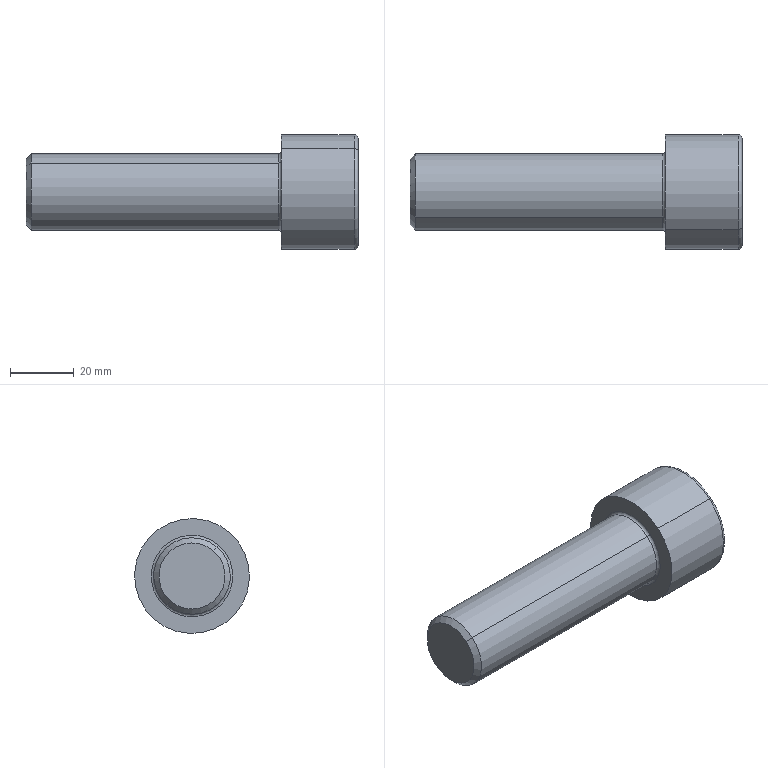Component | SolidWorks | socket head cap screw_iso-3 | 1 solid | 27 faces | box 104 x 36 x 36 mm | volume 55912 mm3 | plane 15 | cone 4 | torus 4 | cylinder 4 | commonest cylinder face diameters 24 x2 36 x2
STEP:
#1=COLOUR_RGB('',0.7922,0.8196,0.9333);
#2=FILL_AREA_STYLE_COLOUR('',#1);
#3=FILL_AREA_STYLE('',(#2));
#4=SURFACE_STYLE_FILL_AREA(#3);
#5=SURFACE_SIDE_STYLE('',(#4));
#6=SURFACE_STYLE_USAGE(.BOTH.,#5);
#7=PRESENTATION_STYLE_ASSIGNMENT((#6));
#8=CARTESIAN_POINT('',(-2.092,1.23,0.6693));
#9=VERTEX_POINT('',#8);
#10=CARTESIAN_POINT('',(-1.873,1.478,0.3823));
#11=VERTEX_POINT('',#10);
#12=CARTESIAN_POINT('',(-1.873,1.478,0.3823));
#13=DIRECTION('',(0.5,0.5664,-0.6551));
#14=VECTOR('',#13,39.37);
#15=LINE('',#12,#14);
#16=EDGE_CURVE('',#9,#11,#15,.T.);
#17=ORIENTED_EDGE('',*,*,#16,.F.);
#18=CARTESIAN_POINT('',(-1.873,0.9822,0.9563));
#19=VERTEX_POINT('',#18);
#20=CARTESIAN_POINT('',(-1.873,0.9822,0.9563));
#21=DIRECTION('',(0.5,-0.5664,0.6551));
#22=VECTOR('',#21,39.37);
#23=LINE('',#20,#22);
#24=EDGE_CURVE('',#9,#19,#23,.T.);
#25=ORIENTED_EDGE('',*,*,#24,.T.);
#26=CARTESIAN_POINT('',(-1.873,0.8577,0.5979));
#27=VERTEX_POINT('',#26);
#28=CARTESIAN_POINT('',(-1.873,1.23,0.6693));
#29=DIRECTION('',(1.,0.,-0.));
#30=DIRECTION('',(0.,0.654,-0.7565));
#31=AXIS2_PLACEMENT_3D('',#28,#29,#30);
#32=CIRCLE('',#31,0.3794);
#33=EDGE_CURVE('',#19,#27,#32,.T.);
#34=ORIENTED_EDGE('',*,*,#33,.T.);
#35=CARTESIAN_POINT('',(-1.873,1.106,0.3109));
#36=VERTEX_POINT('',#35);
#37=CARTESIAN_POINT('',(-1.873,1.23,0.6693));
#38=DIRECTION('',(1.,0.,-0.));
#39=DIRECTION('',(0.,0.654,-0.7565));
#40=AXIS2_PLACEMENT_3D('',#37,#38,#39);
#41=CIRCLE('',#40,0.3794);
#42=EDGE_CURVE('',#27,#36,#41,.T.);
#43=ORIENTED_EDGE('',*,*,#42,.T.);
#44=CARTESIAN_POINT('',(-1.873,1.23,0.6693));
#45=DIRECTION('',(1.,0.,-0.));
#46=DIRECTION('',(0.,0.654,-0.7565));
#47=AXIS2_PLACEMENT_3D('',#44,#45,#46);
#48=CIRCLE('',#47,0.3794);
#49=EDGE_CURVE('',#36,#11,#48,.T.);
#50=ORIENTED_EDGE('',*,*,#49,.T.);
#51=EDGE_LOOP('',(#17,#25,#34,#43,#50));
#52=FACE_OUTER_BOUND('',#51,.T.);
#53=CARTESIAN_POINT('',(-1.873,1.23,0.6693));
#54=DIRECTION('',(1.,0.,-0.));
#55=DIRECTION('',(0.,0.654,-0.7565));
#56=AXIS2_PLACEMENT_3D('',#53,#54,#55);
#57=CONICAL_SURFACE('',#56,0.3794,1.047);
#58=ADVANCED_FACE('',(#52),#57,.F.);
#59=CARTESIAN_POINT('',(-1.425,0.7668,1.205));
#60=VERTEX_POINT('',#59);
#61=CARTESIAN_POINT('',(-1.425,1.694,0.1332));
#62=VERTEX_POINT('',#61);
#63=CARTESIAN_POINT('',(-1.425,1.23,0.6693));
#64=DIRECTION('',(-1.,-0.,0.));
#65=DIRECTION('',(0.,0.654,-0.7565));
#66=AXIS2_PLACEMENT_3D('',#63,#64,#65);
#67=CIRCLE('',#66,0.7087);
#68=EDGE_CURVE('',#60,#62,#67,.T.);
#69=ORIENTED_EDGE('',*,*,#68,.F.);
#70=CARTESIAN_POINT('',(-1.378,0.7977,1.17));
#71=VERTEX_POINT('',#70);
#72=CARTESIAN_POINT('',(-1.425,0.7977,1.17));
#73=DIRECTION('',(-0.,0.7565,0.654));
#74=DIRECTION('',(0.,-0.654,0.7565));
#75=AXIS2_PLACEMENT_3D('',#72,#73,#74);
#76=CIRCLE('',#75,0.04724);
#77=EDGE_CURVE('',#60,#71,#76,.T.);
#78=ORIENTED_EDGE('',*,*,#77,.T.);
#79=CARTESIAN_POINT('',(-1.378,1.663,0.169));
#80=VERTEX_POINT('',#79);
#81=CARTESIAN_POINT('',(-1.378,1.23,0.6693));
#82=DIRECTION('',(1.,0.,-0.));
#83=DIRECTION('',(0.,0.654,-0.7565));
#84=AXIS2_PLACEMENT_3D('',#81,#82,#83);
#85=CIRCLE('',#84,0.6614);
#86=EDGE_CURVE('',#80,#71,#85,.T.);
#87=ORIENTED_EDGE('',*,*,#86,.F.);
#88=CARTESIAN_POINT('',(-1.425,1.663,0.169));
#89=DIRECTION('',(0.,-0.7565,-0.654));
#90=DIRECTION('',(0.,0.654,-0.7565));
#91=AXIS2_PLACEMENT_3D('',#88,#89,#90);
#92=CIRCLE('',#91,0.04724);
#93=EDGE_CURVE('',#62,#80,#92,.T.);
#94=ORIENTED_EDGE('',*,*,#93,.F.);
#95=EDGE_LOOP('',(#69,#78,#87,#94));
#96=FACE_OUTER_BOUND('',#95,.T.);
#97=CARTESIAN_POINT('',(-1.425,1.23,0.6693));
#98=DIRECTION('',(1.,0.,-0.));
#99=DIRECTION('',(-0.,0.654,-0.7565));
#100=AXIS2_PLACEMENT_3D('',#97,#98,#99);
#101=TOROIDAL_SURFACE('',#100,0.6614,0.04724);
#102=ADVANCED_FACE('',(#96),#101,.T.);
#103=CARTESIAN_POINT('',(-2.354,1.539,0.3119));
#104=VERTEX_POINT('',#103);
#105=CARTESIAN_POINT('',(-2.354,0.9213,1.027));
#106=VERTEX_POINT('',#105);
#107=CARTESIAN_POINT('',(-2.354,1.23,0.6693));
#108=DIRECTION('',(-1.,-0.,0.));
#109=DIRECTION('',(0.,-0.654,0.7565));
#110=AXIS2_PLACEMENT_3D('',#107,#108,#109);
#111=CIRCLE('',#110,0.4724);
#112=EDGE_CURVE('',#104,#106,#111,.T.);
#113=ORIENTED_EDGE('',*,*,#112,.F.);
#114=CARTESIAN_POINT('',(-2.323,1.56,0.2881));
#115=VERTEX_POINT('',#114);
#116=CARTESIAN_POINT('',(-2.354,1.56,0.2881));
#117=DIRECTION('',(-0.,0.7565,0.654));
#118=DIRECTION('',(0.,-0.654,0.7565));
#119=AXIS2_PLACEMENT_3D('',#116,#117,#118);
#120=CIRCLE('',#119,0.0315);
#121=EDGE_CURVE('',#104,#115,#120,.T.);
#122=ORIENTED_EDGE('',*,*,#121,.T.);
#123=CARTESIAN_POINT('',(-2.323,0.9007,1.051));
#124=VERTEX_POINT('',#123);
#125=CARTESIAN_POINT('',(-2.323,1.23,0.6693));
#126=DIRECTION('',(1.,0.,-0.));
#127=DIRECTION('',(0.,-0.654,0.7565));
#128=AXIS2_PLACEMENT_3D('',#125,#126,#127);
#129=CIRCLE('',#128,0.5039);
#130=EDGE_CURVE('',#124,#115,#129,.T.);
#131=ORIENTED_EDGE('',*,*,#130,.F.);
#132=CARTESIAN_POINT('',(-2.354,0.9007,1.051));
#133=DIRECTION('',(0.,-0.7565,-0.654));
#134=DIRECTION('',(0.,0.654,-0.7565));
#135=AXIS2_PLACEMENT_3D('',#132,#133,#134);
#136=CIRCLE('',#135,0.0315);
#137=EDGE_CURVE('',#106,#124,#136,.T.);
#138=ORIENTED_EDGE('',*,*,#137,.F.);
#139=EDGE_LOOP('',(#113,#122,#131,#138));
#140=FACE_OUTER_BOUND('',#139,.T.);
#141=CARTESIAN_POINT('',(-2.354,1.23,0.6693));
#142=DIRECTION('',(-1.,-0.,0.));
#143=DIRECTION('',(0.,-0.654,0.7565));
#144=AXIS2_PLACEMENT_3D('',#141,#142,#143);
#145=TOROIDAL_SURFACE('',#144,0.5039,0.0315);
#146=ADVANCED_FACE('',(#140),#145,.F.);
#147=CARTESIAN_POINT('',(-5.472,1.497,0.361));
#148=VERTEX_POINT('',#147);
#149=CARTESIAN_POINT('',(-5.472,0.9638,0.9776));
#150=VERTEX_POINT('',#149);
#151=CARTESIAN_POINT('',(-5.472,1.23,0.6693));
#152=DIRECTION('',(1.,0.,-0.));
#153=DIRECTION('',(0.,0.654,-0.7565));
#154=AXIS2_PLACEMENT_3D('',#151,#152,#153);
#155=CIRCLE('',#154,0.4076);
#156=EDGE_CURVE('',#148,#150,#155,.T.);
#157=ORIENTED_EDGE('',*,*,#156,.T.);
#158=CARTESIAN_POINT('',(-5.408,0.9213,1.027));
#159=VERTEX_POINT('',#158);
#160=CARTESIAN_POINT('',(-5.472,0.9638,0.9776));
#161=DIRECTION('',(0.7071,-0.4625,0.5349));
#162=VECTOR('',#161,39.37);
#163=LINE('',#160,#162);
#164=EDGE_CURVE('',#150,#159,#163,.T.);
#165=ORIENTED_EDGE('',*,*,#164,.T.);
#166=CARTESIAN_POINT('',(-5.408,1.539,0.3119));
#167=VERTEX_POINT('',#166);
#168=CARTESIAN_POINT('',(-5.408,1.23,0.6693));
#169=DIRECTION('',(1.,0.,-0.));
#170=DIRECTION('',(0.,0.654,-0.7565));
#171=AXIS2_PLACEMENT_3D('',#168,#169,#170);
#172=CIRCLE('',#171,0.4724);
#173=EDGE_CURVE('',#167,#159,#172,.T.);
#174=ORIENTED_EDGE('',*,*,#173,.F.);
#175=CARTESIAN_POINT('',(-5.472,1.497,0.361));
#176=DIRECTION('',(0.7071,0.4625,-0.5349));
#177=VECTOR('',#176,39.37);
#178=LINE('',#175,#177);
#179=EDGE_CURVE('',#148,#167,#178,.T.);
#180=ORIENTED_EDGE('',*,*,#179,.F.);
#181=EDGE_LOOP('',(#157,#165,#174,#180));
#182=FACE_OUTER_BOUND('',#181,.T.);
#183=CARTESIAN_POINT('',(-5.472,1.23,0.6693));
#184=DIRECTION('',(1.,0.,-0.));
#185=DIRECTION('',(0.,0.654,-0.7565));
#186=AXIS2_PLACEMENT_3D('',#183,#184,#185);
#187=CONICAL_SURFACE('',#186,0.4076,0.7854);
#188=ADVANCED_FACE('',(#182),#187,.T.);
#189=ORIENTED_EDGE('',*,*,#173,.T.);
#190=CARTESIAN_POINT('',(-0.128,0.9213,1.027));
#191=DIRECTION('',(1.,0.,-0.));
#192=VECTOR('',#191,39.37);
#193=LINE('',#190,#192);
#194=EDGE_CURVE('',#159,#106,#193,.T.);
#195=ORIENTED_EDGE('',*,*,#194,.T.);
#196=CARTESIAN_POINT('',(-2.354,1.23,0.6693));
#197=DIRECTION('',(-1.,-0.,0.));
#198=DIRECTION('',(0.,-0.654,0.7565));
#199=AXIS2_PLACEMENT_3D('',#196,#197,#198);
#200=CIRCLE('',#199,0.4724);
#201=EDGE_CURVE('',#106,#104,#200,.T.);
#202=ORIENTED_EDGE('',*,*,#201,.T.);
#203=CARTESIAN_POINT('',(-0.128,1.539,0.3119));
#204=DIRECTION('',(1.,0.,-0.));
#205=VECTOR('',#204,39.37);
#206=LINE('',#203,#205);
#207=EDGE_CURVE('',#167,#104,#206,.T.);
#208=ORIENTED_EDGE('',*,*,#207,.F.);
#209=EDGE_LOOP('',(#189,#195,#202,#208));
#210=FACE_OUTER_BOUND('',#209,.T.);
#211=CARTESIAN_POINT('',(-0.128,1.23,0.6693));
#212=DIRECTION('',(1.,0.,-0.));
#213=DIRECTION('',(0.,0.654,-0.7565));
#214=AXIS2_PLACEMENT_3D('',#211,#212,#213);
#215=CYLINDRICAL_SURFACE('',#214,0.4724);
#216=ADVANCED_FACE('',(#210),#215,.T.);
#217=CARTESIAN_POINT('',(-2.323,1.694,0.1332));
#218=VERTEX_POINT('',#217);
#219=CARTESIAN_POINT('',(-2.323,0.7668,1.205));
#220=VERTEX_POINT('',#219);
#221=CARTESIAN_POINT('',(-2.323,1.23,0.6693));
#222=DIRECTION('',(1.,0.,-0.));
#223=DIRECTION('',(0.,0.654,-0.7565));
#224=AXIS2_PLACEMENT_3D('',#221,#222,#223);
#225=CIRCLE('',#224,0.7087);
#226=EDGE_CURVE('',#218,#220,#225,.T.);
#227=ORIENTED_EDGE('',*,*,#226,.T.);
#228=CARTESIAN_POINT('',(-0.128,0.7668,1.205));
#229=DIRECTION('',(1.,0.,-0.));
#230=VECTOR('',#229,39.37);
#231=LINE('',#228,#230);
#232=EDGE_CURVE('',#220,#60,#231,.T.);
#233=ORIENTED_EDGE('',*,*,#232,.T.);
#234=ORIENTED_EDGE('',*,*,#68,.T.);
#235=CARTESIAN_POINT('',(-0.128,1.694,0.1332));
#236=DIRECTION('',(1.,0.,-0.));
#237=VECTOR('',#236,39.37);
#238=LINE('',#235,#237);
#239=EDGE_CURVE('',#218,#62,#238,.T.);
#240=ORIENTED_EDGE('',*,*,#239,.F.);
#241=EDGE_LOOP('',(#227,#233,#234,#240));
#242=FACE_OUTER_BOUND('',#241,.T.);
#243=CARTESIAN_POINT('',(-0.128,1.23,0.6693));
#244=DIRECTION('',(1.,0.,-0.));
#245=DIRECTION('',(0.,0.654,-0.7565));
#246=AXIS2_PLACEMENT_3D('',#243,#244,#245);
#247=CYLINDRICAL_SURFACE('',#246,0.7087);
#248=ADVANCED_FACE('',(#242),#247,.T.);
#249=CARTESIAN_POINT('',(-1.378,1.562,0.9558));
#250=VERTEX_POINT('',#249);
#251=CARTESIAN_POINT('',(-1.378,1.644,0.5255));
#252=VERTEX_POINT('',#251);
#253=CARTESIAN_POINT('',(-1.378,1.562,0.9558));
#254=DIRECTION('',(-0.,0.1882,-0.9821));
#255=VECTOR('',#254,39.37);
#256=LINE('',#253,#255);
#257=EDGE_CURVE('',#250,#252,#256,.T.);
#258=ORIENTED_EDGE('',*,*,#257,.T.);
#259=CARTESIAN_POINT('',(-1.378,1.313,0.239));
#260=VERTEX_POINT('',#259);
#261=CARTESIAN_POINT('',(-1.378,1.313,0.239));
#262=DIRECTION('',(-0.,0.7565,0.654));
#263=VECTOR('',#262,39.37);
#264=LINE('',#261,#263);
#265=EDGE_CURVE('',#260,#252,#264,.T.);
#266=ORIENTED_EDGE('',*,*,#265,.F.);
#267=CARTESIAN_POINT('',(-1.378,0.8989,0.3827));
#268=VERTEX_POINT('',#267);
#269=CARTESIAN_POINT('',(-1.378,1.313,0.239));
#270=DIRECTION('',(0.,-0.9446,0.3281));
#271=VECTOR('',#270,39.37);
#272=LINE('',#269,#271);
#273=EDGE_CURVE('',#260,#268,#272,.T.);
#274=ORIENTED_EDGE('',*,*,#273,.T.);
#275=CARTESIAN_POINT('',(-1.378,0.8164,0.813));
#276=VERTEX_POINT('',#275);
#277=CARTESIAN_POINT('',(-1.378,0.8989,0.3827));
#278=DIRECTION('',(0.,-0.1882,0.9821));
#279=VECTOR('',#278,39.37);
#280=LINE('',#277,#279);
#281=EDGE_CURVE('',#268,#276,#280,.T.);
#282=ORIENTED_EDGE('',*,*,#281,.T.);
#283=CARTESIAN_POINT('',(-1.378,1.148,1.1));
#284=VERTEX_POINT('',#283);
#285=CARTESIAN_POINT('',(-1.378,1.148,1.1));
#286=DIRECTION('',(0.,-0.7565,-0.654));
#287=VECTOR('',#286,39.37);
#288=LINE('',#285,#287);
#289=EDGE_CURVE('',#284,#276,#288,.T.);
#290=ORIENTED_EDGE('',*,*,#289,.F.);
#291=CARTESIAN_POINT('',(-1.378,1.562,0.9558));
#292=DIRECTION('',(0.,-0.9446,0.3281));
#293=VECTOR('',#292,39.37);
#294=LINE('',#291,#293);
#295=EDGE_CURVE('',#250,#284,#294,.T.);
#296=ORIENTED_EDGE('',*,*,#295,.F.);
#297=EDGE_LOOP('',(#258,#266,#274,#282,#290,#296));
#298=FACE_BOUND('',#297,.T.);
#299=ORIENTED_EDGE('',*,*,#86,.T.);
#300=CARTESIAN_POINT('',(-1.378,1.23,0.6693));
#301=DIRECTION('',(1.,0.,-0.));
#302=DIRECTION('',(0.,0.654,-0.7565));
#303=AXIS2_PLACEMENT_3D('',#300,#301,#302);
#304=CIRCLE('',#303,0.6614);
#305=EDGE_CURVE('',#71,#80,#304,.T.);
#306=ORIENTED_EDGE('',*,*,#305,.T.);
#307=EDGE_LOOP('',(#299,#306));
#308=FACE_OUTER_BOUND('',#307,.T.);
#309=CARTESIAN_POINT('',(-1.378,1.23,0.6693));
#310=DIRECTION('',(1.,0.,0.));
#311=DIRECTION('',(-0.,0.654,-0.7565));
#312=AXIS2_PLACEMENT_3D('',#309,#310,#311);
#313=PLANE('',#312);
#314=ADVANCED_FACE('',(#298,#308),#313,.T.);
#315=ORIENTED_EDGE('',*,*,#232,.F.);
#316=CARTESIAN_POINT('',(-2.323,1.23,0.6693));
#317=DIRECTION('',(1.,0.,-0.));
#318=DIRECTION('',(0.,0.654,-0.7565));
#319=AXIS2_PLACEMENT_3D('',#316,#317,#318);
#320=CIRCLE('',#319,0.7087);
#321=EDGE_CURVE('',#220,#218,#320,.T.);
#322=ORIENTED_EDGE('',*,*,#321,.T.);
#323=ORIENTED_EDGE('',*,*,#239,.T.);
#324=CARTESIAN_POINT('',(-1.425,1.23,0.6693));
#325=DIRECTION('',(-1.,-0.,0.));
#326=DIRECTION('',(0.,0.654,-0.7565));
#327=AXIS2_PLACEMENT_3D('',#324,#325,#326);
#328=CIRCLE('',#327,0.7087);
#329=EDGE_CURVE('',#62,#60,#328,.T.);
#330=ORIENTED_EDGE('',*,*,#329,.T.);
#331=EDGE_LOOP('',(#315,#322,#323,#330));
#332=FACE_OUTER_BOUND('',#331,.T.);
#333=CARTESIAN_POINT('',(-0.128,1.23,0.6693));
#334=DIRECTION('',(1.,0.,-0.));
#335=DIRECTION('',(0.,0.654,-0.7565));
#336=AXIS2_PLACEMENT_3D('',#333,#334,#335);
#337=CYLINDRICAL_SURFACE('',#336,0.7087);
#338=ADVANCED_FACE('',(#332),#337,.T.);
#339=ORIENTED_EDGE('',*,*,#130,.T.);
#340=CARTESIAN_POINT('',(-2.323,1.23,0.6693));
#341=DIRECTION('',(1.,0.,-0.));
#342=DIRECTION('',(0.,-0.654,0.7565));
#343=AXIS2_PLACEMENT_3D('',#340,#341,#342);
#344=CIRCLE('',#343,0.5039);
#345=EDGE_CURVE('',#115,#124,#344,.T.);
#346=ORIENTED_EDGE('',*,*,#345,.T.);
#347=EDGE_LOOP('',(#339,#346));
#348=FACE_BOUND('',#347,.T.);
#349=ORIENTED_EDGE('',*,*,#226,.F.);
#350=ORIENTED_EDGE('',*,*,#321,.F.);
#351=EDGE_LOOP('',(#349,#350));
#352=FACE_OUTER_BOUND('',#351,.T.);
#353=CARTESIAN_POINT('',(-2.323,1.766,1.133));
#354=DIRECTION('',(-1.,-0.,0.));
#355=DIRECTION('',(0.,-0.654,0.7565));
#356=AXIS2_PLACEMENT_3D('',#353,#354,#355);
#357=PLANE('',#356);
#358=ADVANCED_FACE('',(#348,#352),#357,.T.);
#359=ORIENTED_EDGE('',*,*,#194,.F.);
#360=CARTESIAN_POINT('',(-5.408,1.23,0.6693));
#361=DIRECTION('',(1.,0.,-0.));
#362=DIRECTION('',(0.,0.654,-0.7565));
#363=AXIS2_PLACEMENT_3D('',#360,#361,#362);
#364=CIRCLE('',#363,0.4724);
#365=EDGE_CURVE('',#159,#167,#364,.T.);
#366=ORIENTED_EDGE('',*,*,#365,.T.);
#367=ORIENTED_EDGE('',*,*,#207,.T.);
#368=ORIENTED_EDGE('',*,*,#112,.T.);
#369=EDGE_LOOP('',(#359,#366,#367,#368));
#370=FACE_OUTER_BOUND('',#369,.T.);
#371=CARTESIAN_POINT('',(-0.128,1.23,0.6693));
#372=DIRECTION('',(1.,0.,-0.));
#373=DIRECTION('',(0.,0.654,-0.7565));
#374=AXIS2_PLACEMENT_3D('',#371,#372,#373);
#375=CYLINDRICAL_SURFACE('',#374,0.4724);
#376=ADVANCED_FACE('',(#370),#375,.T.);
#377=ORIENTED_EDGE('',*,*,#164,.F.);
#378=CARTESIAN_POINT('',(-5.472,1.23,0.6693));
#379=DIRECTION('',(1.,0.,-0.));
#380=DIRECTION('',(0.,0.654,-0.7565));
#381=AXIS2_PLACEMENT_3D('',#378,#379,#380);
#382=CIRCLE('',#381,0.4076);
#383=EDGE_CURVE('',#150,#148,#382,.T.);
#384=ORIENTED_EDGE('',*,*,#383,.T.);
#385=ORIENTED_EDGE('',*,*,#179,.T.);
#386=ORIENTED_EDGE('',*,*,#365,.F.);
#387=EDGE_LOOP('',(#377,#384,#385,#386));
#388=FACE_OUTER_BOUND('',#387,.T.);
#389=CARTESIAN_POINT('',(-5.472,1.23,0.6693));
#390=DIRECTION('',(1.,0.,-0.));
#391=DIRECTION('',(0.,0.654,-0.7565));
#392=AXIS2_PLACEMENT_3D('',#389,#390,#391);
#393=CONICAL_SURFACE('',#392,0.4076,0.7854);
#394=ADVANCED_FACE('',(#388),#393,.T.);
#395=ORIENTED_EDGE('',*,*,#156,.F.);
#396=ORIENTED_EDGE('',*,*,#383,.F.);
#397=EDGE_LOOP('',(#395,#396));
#398=FACE_OUTER_BOUND('',#397,.T.);
#399=CARTESIAN_POINT('',(-5.472,1.539,0.9358));
#400=DIRECTION('',(-1.,-0.,0.));
#401=DIRECTION('',(0.,-0.654,0.7565));
#402=AXIS2_PLACEMENT_3D('',#399,#400,#401);
#403=PLANE('',#402);
#404=ADVANCED_FACE('',(#398),#403,.T.);
#405=ORIENTED_EDGE('',*,*,#121,.F.);
#406=ORIENTED_EDGE('',*,*,#201,.F.);
#407=ORIENTED_EDGE('',*,*,#137,.T.);
#408=ORIENTED_EDGE('',*,*,#345,.F.);
#409=EDGE_LOOP('',(#405,#406,#407,#408));
#410=FACE_OUTER_BOUND('',#409,.T.);
#411=CARTESIAN_POINT('',(-2.354,1.23,0.6693));
#412=DIRECTION('',(-1.,-0.,0.));
#413=DIRECTION('',(0.,-0.654,0.7565));
#414=AXIS2_PLACEMENT_3D('',#411,#412,#413);
#415=TOROIDAL_SURFACE('',#414,0.5039,0.0315);
#416=ADVANCED_FACE('',(#410),#415,.F.);
#417=ORIENTED_EDGE('',*,*,#77,.F.);
#418=ORIENTED_EDGE('',*,*,#329,.F.);
#419=ORIENTED_EDGE('',*,*,#93,.T.);
#420=ORIENTED_EDGE('',*,*,#305,.F.);
#421=EDGE_LOOP('',(#417,#418,#419,#420));
#422=FACE_OUTER_BOUND('',#421,.T.);
#423=CARTESIAN_POINT('',(-1.425,1.23,0.6693));
#424=DIRECTION('',(1.,0.,-0.));
#425=DIRECTION('',(-0.,0.654,-0.7565));
#426=AXIS2_PLACEMENT_3D('',#423,#424,#425);
#427=TOROIDAL_SURFACE('',#426,0.6614,0.04724);
#428=ADVANCED_FACE('',(#422),#427,.T.);
#429=ORIENTED_EDGE('',*,*,#257,.F.);
#430=CARTESIAN_POINT('',(-1.873,1.562,0.9558));
#431=VERTEX_POINT('',#430);
#432=CARTESIAN_POINT('',(-1.873,1.562,0.9558));
#433=DIRECTION('',(1.,0.,-0.));
#434=VECTOR('',#433,39.37);
#435=LINE('',#432,#434);
#436=EDGE_CURVE('',#431,#250,#435,.T.);
#437=ORIENTED_EDGE('',*,*,#436,.F.);
#438=CARTESIAN_POINT('',(-1.873,1.603,0.7407));
#439=VERTEX_POINT('',#438);
#440=CARTESIAN_POINT('',(-1.873,1.562,0.9558));
#441=DIRECTION('',(-0.,0.1882,-0.9821));
#442=VECTOR('',#441,39.37);
#443=LINE('',#440,#442);
#444=EDGE_CURVE('',#431,#439,#443,.T.);
#445=ORIENTED_EDGE('',*,*,#444,.T.);
#446=CARTESIAN_POINT('',(-1.873,1.644,0.5255));
#447=VERTEX_POINT('',#446);
#448=CARTESIAN_POINT('',(-1.873,1.562,0.9558));
#449=DIRECTION('',(-0.,0.1882,-0.9821));
#450=VECTOR('',#449,39.37);
#451=LINE('',#448,#450);
#452=EDGE_CURVE('',#439,#447,#451,.T.);
#453=ORIENTED_EDGE('',*,*,#452,.T.);
#454=CARTESIAN_POINT('',(-1.873,1.644,0.5255));
#455=DIRECTION('',(1.,0.,-0.));
#456=VECTOR('',#455,39.37);
#457=LINE('',#454,#456);
#458=EDGE_CURVE('',#447,#252,#457,.T.);
#459=ORIENTED_EDGE('',*,*,#458,.T.);
#460=EDGE_LOOP('',(#429,#437,#445,#453,#459));
#461=FACE_OUTER_BOUND('',#460,.T.);
#462=CARTESIAN_POINT('',(-1.873,1.562,0.9558));
#463=DIRECTION('',(0.,-0.9821,-0.1882));
#464=DIRECTION('',(0.,-0.1882,0.9821));
#465=AXIS2_PLACEMENT_3D('',#462,#463,#464);
#466=PLANE('',#465);
#467=ADVANCED_FACE('',(#461),#466,.T.);
#468=ORIENTED_EDGE('',*,*,#265,.T.);
#469=ORIENTED_EDGE('',*,*,#458,.F.);
#470=CARTESIAN_POINT('',(-1.873,1.313,0.239));
#471=DIRECTION('',(-0.,0.7565,0.654));
#472=VECTOR('',#471,39.37);
#473=LINE('',#470,#472);
#474=EDGE_CURVE('',#11,#447,#473,.T.);
#475=ORIENTED_EDGE('',*,*,#474,.F.);
#476=CARTESIAN_POINT('',(-1.873,1.313,0.239));
#477=VERTEX_POINT('',#476);
#478=CARTESIAN_POINT('',(-1.873,1.313,0.239));
#479=DIRECTION('',(-0.,0.7565,0.654));
#480=VECTOR('',#479,39.37);
#481=LINE('',#478,#480);
#482=EDGE_CURVE('',#477,#11,#481,.T.);
#483=ORIENTED_EDGE('',*,*,#482,.F.);
#484=CARTESIAN_POINT('',(-1.873,1.313,0.239));
#485=DIRECTION('',(1.,0.,-0.));
#486=VECTOR('',#485,39.37);
#487=LINE('',#484,#486);
#488=EDGE_CURVE('',#477,#260,#487,.T.);
#489=ORIENTED_EDGE('',*,*,#488,.T.);
#490=EDGE_LOOP('',(#468,#469,#475,#483,#489));
#491=FACE_OUTER_BOUND('',#490,.T.);
#492=CARTESIAN_POINT('',(-1.873,1.313,0.239));
#493=DIRECTION('',(-0.,0.654,-0.7565));
#494=DIRECTION('',(0.,-0.7565,-0.654));
#495=AXIS2_PLACEMENT_3D('',#492,#493,#494);
#496=PLANE('',#495);
#497=ADVANCED_FACE('',(#491),#496,.F.);
#498=ORIENTED_EDGE('',*,*,#273,.F.);
#499=ORIENTED_EDGE('',*,*,#488,.F.);
#500=CARTESIAN_POINT('',(-1.873,1.313,0.239));
#501=DIRECTION('',(0.,-0.9446,0.3281));
#502=VECTOR('',#501,39.37);
#503=LINE('',#500,#502);
#504=EDGE_CURVE('',#477,#36,#503,.T.);
#505=ORIENTED_EDGE('',*,*,#504,.T.);
#506=CARTESIAN_POINT('',(-1.873,0.8989,0.3827));
#507=VERTEX_POINT('',#506);
#508=CARTESIAN_POINT('',(-1.873,1.313,0.239));
#509=DIRECTION('',(0.,-0.9446,0.3281));
#510=VECTOR('',#509,39.37);
#511=LINE('',#508,#510);
#512=EDGE_CURVE('',#36,#507,#511,.T.);
#513=ORIENTED_EDGE('',*,*,#512,.T.);
#514=CARTESIAN_POINT('',(-1.873,0.8989,0.3827));
#515=DIRECTION('',(1.,0.,-0.));
#516=VECTOR('',#515,39.37);
#517=LINE('',#514,#516);
#518=EDGE_CURVE('',#507,#268,#517,.T.);
#519=ORIENTED_EDGE('',*,*,#518,.T.);
#520=EDGE_LOOP('',(#498,#499,#505,#513,#519));
#521=FACE_OUTER_BOUND('',#520,.T.);
#522=CARTESIAN_POINT('',(-1.873,1.313,0.239));
#523=DIRECTION('',(-0.,0.3281,0.9446));
#524=DIRECTION('',(-0.,0.9446,-0.3281));
#525=AXIS2_PLACEMENT_3D('',#522,#523,#524);
#526=PLANE('',#525);
#527=ADVANCED_FACE('',(#521),#526,.T.);
#528=ORIENTED_EDGE('',*,*,#281,.F.);
#529=ORIENTED_EDGE('',*,*,#518,.F.);
#530=CARTESIAN_POINT('',(-1.873,0.8989,0.3827));
#531=DIRECTION('',(0.,-0.1882,0.9821));
#532=VECTOR('',#531,39.37);
#533=LINE('',#530,#532);
#534=EDGE_CURVE('',#507,#27,#533,.T.);
#535=ORIENTED_EDGE('',*,*,#534,.T.);
#536=CARTESIAN_POINT('',(-1.873,0.8164,0.813));
#537=VERTEX_POINT('',#536);
#538=CARTESIAN_POINT('',(-1.873,0.8989,0.3827));
#539=DIRECTION('',(0.,-0.1882,0.9821));
#540=VECTOR('',#539,39.37);
#541=LINE('',#538,#540);
#542=EDGE_CURVE('',#27,#537,#541,.T.);
#543=ORIENTED_EDGE('',*,*,#542,.T.);
#544=CARTESIAN_POINT('',(-1.873,0.8164,0.813));
#545=DIRECTION('',(1.,0.,-0.));
#546=VECTOR('',#545,39.37);
#547=LINE('',#544,#546);
#548=EDGE_CURVE('',#537,#276,#547,.T.);
#549=ORIENTED_EDGE('',*,*,#548,.T.);
#550=EDGE_LOOP('',(#528,#529,#535,#543,#549));
#551=FACE_OUTER_BOUND('',#550,.T.);
#552=CARTESIAN_POINT('',(-1.873,0.8989,0.3827));
#553=DIRECTION('',(-0.,0.9821,0.1882));
#554=DIRECTION('',(-0.,0.1882,-0.9821));
#555=AXIS2_PLACEMENT_3D('',#552,#553,#554);
#556=PLANE('',#555);
#557=ADVANCED_FACE('',(#551),#556,.T.);
#558=ORIENTED_EDGE('',*,*,#289,.T.);
#559=ORIENTED_EDGE('',*,*,#548,.F.);
#560=CARTESIAN_POINT('',(-1.873,1.148,1.1));
#561=DIRECTION('',(0.,-0.7565,-0.654));
#562=VECTOR('',#561,39.37);
#563=LINE('',#560,#562);
#564=EDGE_CURVE('',#19,#537,#563,.T.);
#565=ORIENTED_EDGE('',*,*,#564,.F.);
#566=CARTESIAN_POINT('',(-1.873,1.148,1.1));
#567=VERTEX_POINT('',#566);
#568=CARTESIAN_POINT('',(-1.873,1.148,1.1));
#569=DIRECTION('',(0.,-0.7565,-0.654));
#570=VECTOR('',#569,39.37);
#571=LINE('',#568,#570);
#572=EDGE_CURVE('',#567,#19,#571,.T.);
#573=ORIENTED_EDGE('',*,*,#572,.F.);
#574=CARTESIAN_POINT('',(-1.873,1.148,1.1));
#575=DIRECTION('',(1.,0.,-0.));
#576=VECTOR('',#575,39.37);
#577=LINE('',#574,#576);
#578=EDGE_CURVE('',#567,#284,#577,.T.);
#579=ORIENTED_EDGE('',*,*,#578,.T.);
#580=EDGE_LOOP('',(#558,#559,#565,#573,#579));
#581=FACE_OUTER_BOUND('',#580,.T.);
#582=CARTESIAN_POINT('',(-1.873,1.148,1.1));
#583=DIRECTION('',(0.,-0.654,0.7565));
#584=DIRECTION('',(-0.,0.7565,0.654));
#585=AXIS2_PLACEMENT_3D('',#582,#583,#584);
#586=PLANE('',#585);
#587=ADVANCED_FACE('',(#581),#586,.F.);
#588=ORIENTED_EDGE('',*,*,#295,.T.);
#589=ORIENTED_EDGE('',*,*,#578,.F.);
#590=CARTESIAN_POINT('',(-1.873,1.355,1.028));
#591=VERTEX_POINT('',#590);
#592=CARTESIAN_POINT('',(-1.873,1.562,0.9558));
#593=DIRECTION('',(0.,-0.9446,0.3281));
#594=VECTOR('',#593,39.37);
#595=LINE('',#592,#594);
#596=EDGE_CURVE('',#591,#567,#595,.T.);
#597=ORIENTED_EDGE('',*,*,#596,.F.);
#598=CARTESIAN_POINT('',(-1.873,1.562,0.9558));
#599=DIRECTION('',(0.,-0.9446,0.3281));
#600=VECTOR('',#599,39.37);
#601=LINE('',#598,#600);
#602=EDGE_CURVE('',#431,#591,#601,.T.);
#603=ORIENTED_EDGE('',*,*,#602,.F.);
#604=ORIENTED_EDGE('',*,*,#436,.T.);
#605=EDGE_LOOP('',(#588,#589,#597,#603,#604));
#606=FACE_OUTER_BOUND('',#605,.T.);
#607=CARTESIAN_POINT('',(-1.873,1.562,0.9558));
#608=DIRECTION('',(-0.,0.3281,0.9446));
#609=DIRECTION('',(-0.,0.9446,-0.3281));
#610=AXIS2_PLACEMENT_3D('',#607,#608,#609);
#611=PLANE('',#610);
#612=ADVANCED_FACE('',(#606),#611,.F.);
#613=ORIENTED_EDGE('',*,*,#49,.F.);
#614=ORIENTED_EDGE('',*,*,#504,.F.);
#615=ORIENTED_EDGE('',*,*,#482,.T.);
#616=EDGE_LOOP('',(#613,#614,#615));
#617=FACE_OUTER_BOUND('',#616,.T.);
#618=CARTESIAN_POINT('',(-1.873,1.644,0.5255));
#619=DIRECTION('',(1.,0.,0.));
#620=DIRECTION('',(-0.,0.654,-0.7565));
#621=AXIS2_PLACEMENT_3D('',#618,#619,#620);
#622=PLANE('',#621);
#623=ADVANCED_FACE('',(#617),#622,.T.);
#624=ORIENTED_EDGE('',*,*,#42,.F.);
#625=ORIENTED_EDGE('',*,*,#534,.F.);
#626=ORIENTED_EDGE('',*,*,#512,.F.);
#627=EDGE_LOOP('',(#624,#625,#626));
#628=FACE_OUTER_BOUND('',#627,.T.);
#629=CARTESIAN_POINT('',(-1.873,1.644,0.5255));
#630=DIRECTION('',(1.,0.,0.));
#631=DIRECTION('',(-0.,0.654,-0.7565));
#632=AXIS2_PLACEMENT_3D('',#629,#630,#631);
#633=PLANE('',#632);
#634=ADVANCED_FACE('',(#628),#633,.T.);
#635=ORIENTED_EDGE('',*,*,#33,.F.);
#636=ORIENTED_EDGE('',*,*,#564,.T.);
#637=ORIENTED_EDGE('',*,*,#542,.F.);
#638=EDGE_LOOP('',(#635,#636,#637));
#639=FACE_OUTER_BOUND('',#638,.T.);
#640=CARTESIAN_POINT('',(-1.873,1.644,0.5255));
#641=DIRECTION('',(1.,0.,0.));
#642=DIRECTION('',(-0.,0.654,-0.7565));
#643=AXIS2_PLACEMENT_3D('',#640,#641,#642);
#644=PLANE('',#643);
#645=ADVANCED_FACE('',(#639),#644,.T.);
#646=CARTESIAN_POINT('',(-1.873,1.23,0.6693));
#647=DIRECTION('',(1.,0.,-0.));
#648=DIRECTION('',(0.,0.654,-0.7565));
#649=AXIS2_PLACEMENT_3D('',#646,#647,#648);
#650=CIRCLE('',#649,0.3794);
#651=EDGE_CURVE('',#591,#19,#650,.T.);
#652=ORIENTED_EDGE('',*,*,#651,.F.);
#653=ORIENTED_EDGE('',*,*,#596,.T.);
#654=ORIENTED_EDGE('',*,*,#572,.T.);
#655=EDGE_LOOP('',(#652,#653,#654));
#656=FACE_OUTER_BOUND('',#655,.T.);
#657=CARTESIAN_POINT('',(-1.873,1.644,0.5255));
#658=DIRECTION('',(1.,0.,0.));
#659=DIRECTION('',(-0.,0.654,-0.7565));
#660=AXIS2_PLACEMENT_3D('',#657,#658,#659);
#661=PLANE('',#660);
#662=ADVANCED_FACE('',(#656),#661,.T.);
#663=CARTESIAN_POINT('',(-1.873,1.23,0.6693));
#664=DIRECTION('',(1.,0.,-0.));
#665=DIRECTION('',(0.,0.654,-0.7565));
#666=AXIS2_PLACEMENT_3D('',#663,#664,#665);
#667=CIRCLE('',#666,0.3794);
#668=EDGE_CURVE('',#439,#591,#667,.T.);
#669=ORIENTED_EDGE('',*,*,#668,.F.);
#670=ORIENTED_EDGE('',*,*,#444,.F.);
#671=ORIENTED_EDGE('',*,*,#602,.T.);
#672=EDGE_LOOP('',(#669,#670,#671));
#673=FACE_OUTER_BOUND('',#672,.T.);
#674=CARTESIAN_POINT('',(-1.873,1.644,0.5255));
#675=DIRECTION('',(1.,0.,0.));
#676=DIRECTION('',(-0.,0.654,-0.7565));
#677=AXIS2_PLACEMENT_3D('',#674,#675,#676);
#678=PLANE('',#677);
#679=ADVANCED_FACE('',(#673),#678,.T.);
#680=CARTESIAN_POINT('',(-1.873,1.23,0.6693));
#681=DIRECTION('',(1.,0.,-0.));
#682=DIRECTION('',(0.,0.654,-0.7565));
#683=AXIS2_PLACEMENT_3D('',#680,#681,#682);
#684=CIRCLE('',#683,0.3794);
#685=EDGE_CURVE('',#11,#439,#684,.T.);
#686=ORIENTED_EDGE('',*,*,#685,.F.);
#687=ORIENTED_EDGE('',*,*,#474,.T.);
#688=ORIENTED_EDGE('',*,*,#452,.F.);
#689=EDGE_LOOP('',(#686,#687,#688));
#690=FACE_OUTER_BOUND('',#689,.T.);
#691=CARTESIAN_POINT('',(-1.873,1.644,0.5255));
#692=DIRECTION('',(1.,0.,0.));
#693=DIRECTION('',(-0.,0.654,-0.7565));
#694=AXIS2_PLACEMENT_3D('',#691,#692,#693);
#695=PLANE('',#694);
#696=ADVANCED_FACE('',(#690),#695,.T.);
#697=ORIENTED_EDGE('',*,*,#24,.F.);
#698=ORIENTED_EDGE('',*,*,#16,.T.);
#699=ORIENTED_EDGE('',*,*,#685,.T.);
#700=ORIENTED_EDGE('',*,*,#668,.T.);
#701=ORIENTED_EDGE('',*,*,#651,.T.);
#702=EDGE_LOOP('',(#697,#698,#699,#700,#701));
#703=FACE_OUTER_BOUND('',#702,.T.);
#704=CARTESIAN_POINT('',(-1.873,1.23,0.6693));
#705=DIRECTION('',(1.,0.,-0.));
#706=DIRECTION('',(0.,0.654,-0.7565));
#707=AXIS2_PLACEMENT_3D('',#704,#705,#706);
#708=CONICAL_SURFACE('',#707,0.3794,1.047);
#709=ADVANCED_FACE('',(#703),#708,.F.);
#710=CLOSED_SHELL('',(#58,#102,#146,#188,#216,#248,#314,#338,#358,#376,#394,#404,#416,#428,#467,#497,#527,#557,#587,#612,#623,#634,#645,#662,#679,#696,#709));
#711=MANIFOLD_SOLID_BREP('',#710);
#712=STYLED_ITEM('',(#7),#711);
#713=PRESENTATION_LAYER_ASSIGNMENT('','',(#712));
#714=(LENGTH_UNIT()NAMED_UNIT(*)SI_UNIT($,.METRE.));
#715=LENGTH_MEASURE_WITH_UNIT(LENGTH_MEASURE(0.0254),#714);
#716=DIMENSIONAL_EXPONENTS(1.,0.,0.,0.,0.,0.,0.);
#717=(CONVERSION_BASED_UNIT('',#715)LENGTH_UNIT()NAMED_UNIT(#716));
#718=UNCERTAINTY_MEASURE_WITH_UNIT(LENGTH_MEASURE(0.00001),#717,'','');
#719=(NAMED_UNIT(*)PLANE_ANGLE_UNIT()SI_UNIT($,.RADIAN.));
#720=(NAMED_UNIT(*)SI_UNIT($,.STERADIAN.)SOLID_ANGLE_UNIT());
#721=(GEOMETRIC_REPRESENTATION_CONTEXT(3)GLOBAL_UNCERTAINTY_ASSIGNED_CONTEXT((#718))GLOBAL_UNIT_ASSIGNED_CONTEXT((#717,#719,#720))REPRESENTATION_CONTEXT('',''));
#722=MECHANICAL_DESIGN_GEOMETRIC_PRESENTATION_REPRESENTATION('',(#712),#721);
#723=CARTESIAN_POINT('',(0.,0.,0.));
#724=DIRECTION('',(0.,0.,1.));
#725=DIRECTION('',(1.,0.,0.));
#726=AXIS2_PLACEMENT_3D('',#723,#724,#725);
#727=(LENGTH_UNIT()NAMED_UNIT(*)SI_UNIT($,.METRE.));
#728=LENGTH_MEASURE_WITH_UNIT(LENGTH_MEASURE(0.0254),#727);
#729=DIMENSIONAL_EXPONENTS(1.,0.,0.,0.,0.,0.,0.);
#730=(CONVERSION_BASED_UNIT('',#728)LENGTH_UNIT()NAMED_UNIT(#729));
#731=UNCERTAINTY_MEASURE_WITH_UNIT(LENGTH_MEASURE(0.00001),#730,'','');
#732=(NAMED_UNIT(*)PLANE_ANGLE_UNIT()SI_UNIT($,.RADIAN.));
#733=(NAMED_UNIT(*)SI_UNIT($,.STERADIAN.)SOLID_ANGLE_UNIT());
#734=(GEOMETRIC_REPRESENTATION_CONTEXT(3)GLOBAL_UNCERTAINTY_ASSIGNED_CONTEXT((#731))GLOBAL_UNIT_ASSIGNED_CONTEXT((#730,#732,#733))REPRESENTATION_CONTEXT('',''));
#735=ADVANCED_BREP_SHAPE_REPRESENTATION('',(#711,#726),#734);